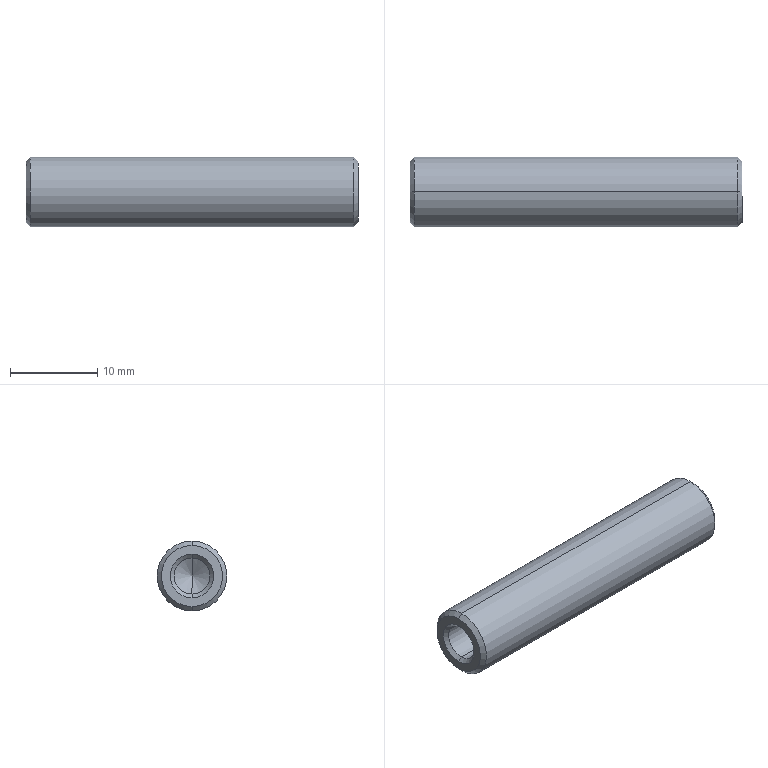Component | SolidWorks | MHF04-D8-L38.stp-1 | 1 solid | 20 faces | box 38 x 8 x 8 mm | volume 1481 mm3 | cone 12 | cylinder 6 | plane 2 | commonest cylinder face diameters 4.134 x4 8 x2
STEP:
#1=CARTESIAN_POINT('',(0.1007,3.568,-1.181));
#2=VERTEX_POINT('',#1);
#3=CARTESIAN_POINT('',(0.1476,3.568,-1.262));
#4=VERTEX_POINT('',#3);
#5=CARTESIAN_POINT('',(0.1476,3.568,-1.262));
#6=DIRECTION('',(0.5,0.,-0.866));
#7=VECTOR('',#6,39.37);
#8=LINE('',#5,#7);
#9=EDGE_CURVE('',#2,#4,#8,.T.);
#10=ORIENTED_EDGE('',*,*,#9,.F.);
#11=CARTESIAN_POINT('',(0.1476,3.568,-1.1));
#12=VERTEX_POINT('',#11);
#13=CARTESIAN_POINT('',(0.1476,3.568,-1.1));
#14=DIRECTION('',(0.5,-0.,0.866));
#15=VECTOR('',#14,39.37);
#16=LINE('',#13,#15);
#17=EDGE_CURVE('',#2,#12,#16,.T.);
#18=ORIENTED_EDGE('',*,*,#17,.T.);
#19=CARTESIAN_POINT('',(0.1476,3.568,-1.181));
#20=DIRECTION('',(1.,0.,0.));
#21=DIRECTION('',(0.,0.,-1.));
#22=AXIS2_PLACEMENT_3D('',#19,#20,#21);
#23=CIRCLE('',#22,0.08138);
#24=EDGE_CURVE('',#12,#4,#23,.T.);
#25=ORIENTED_EDGE('',*,*,#24,.T.);
#26=EDGE_LOOP('',(#10,#18,#25));
#27=FACE_OUTER_BOUND('',#26,.T.);
#28=CARTESIAN_POINT('',(0.1476,3.568,-1.181));
#29=DIRECTION('',(1.,0.,0.));
#30=DIRECTION('',(0.,0.,-1.));
#31=AXIS2_PLACEMENT_3D('',#28,#29,#30);
#32=CONICAL_SURFACE('',#31,0.08138,1.047);
#33=ADVANCED_FACE('',(#27),#32,.F.);
#34=CARTESIAN_POINT('',(0.731,3.568,-1.262));
#35=VERTEX_POINT('',#34);
#36=CARTESIAN_POINT('',(0.731,3.568,-1.1));
#37=VERTEX_POINT('',#36);
#38=CARTESIAN_POINT('',(0.731,3.568,-1.181));
#39=DIRECTION('',(1.,0.,0.));
#40=DIRECTION('',(0.,0.,-1.));
#41=AXIS2_PLACEMENT_3D('',#38,#39,#40);
#42=CIRCLE('',#41,0.08138);
#43=EDGE_CURVE('',#35,#37,#42,.T.);
#44=ORIENTED_EDGE('',*,*,#43,.T.);
#45=CARTESIAN_POINT('',(0.748,3.568,-1.1));
#46=DIRECTION('',(-1.,-0.,-0.));
#47=VECTOR('',#46,39.37);
#48=LINE('',#45,#47);
#49=EDGE_CURVE('',#37,#12,#48,.T.);
#50=ORIENTED_EDGE('',*,*,#49,.T.);
#51=CARTESIAN_POINT('',(0.1476,3.568,-1.181));
#52=DIRECTION('',(1.,0.,0.));
#53=DIRECTION('',(0.,0.,-1.));
#54=AXIS2_PLACEMENT_3D('',#51,#52,#53);
#55=CIRCLE('',#54,0.08138);
#56=EDGE_CURVE('',#4,#12,#55,.T.);
#57=ORIENTED_EDGE('',*,*,#56,.F.);
#58=CARTESIAN_POINT('',(0.748,3.568,-1.262));
#59=DIRECTION('',(-1.,-0.,-0.));
#60=VECTOR('',#59,39.37);
#61=LINE('',#58,#60);
#62=EDGE_CURVE('',#35,#4,#61,.T.);
#63=ORIENTED_EDGE('',*,*,#62,.F.);
#64=EDGE_LOOP('',(#44,#50,#57,#63));
#65=FACE_OUTER_BOUND('',#64,.T.);
#66=CARTESIAN_POINT('',(0.748,3.568,-1.181));
#67=DIRECTION('',(-1.,-0.,-0.));
#68=DIRECTION('',(0.,0.,-1.));
#69=AXIS2_PLACEMENT_3D('',#66,#67,#68);
#70=CYLINDRICAL_SURFACE('',#69,0.08138);
#71=ADVANCED_FACE('',(#65),#70,.F.);
#72=CARTESIAN_POINT('',(0.731,3.568,-1.181));
#73=DIRECTION('',(1.,0.,0.));
#74=DIRECTION('',(0.,0.,-1.));
#75=AXIS2_PLACEMENT_3D('',#72,#73,#74);
#76=CIRCLE('',#75,0.08138);
#77=EDGE_CURVE('',#37,#35,#76,.T.);
#78=ORIENTED_EDGE('',*,*,#77,.F.);
#79=CARTESIAN_POINT('',(0.748,3.568,-1.083));
#80=VERTEX_POINT('',#79);
#81=CARTESIAN_POINT('',(0.748,3.568,-1.083));
#82=DIRECTION('',(0.7071,0.,0.7071));
#83=VECTOR('',#82,39.37);
#84=LINE('',#81,#83);
#85=EDGE_CURVE('',#37,#80,#84,.T.);
#86=ORIENTED_EDGE('',*,*,#85,.T.);
#87=CARTESIAN_POINT('',(0.748,3.568,-1.28));
#88=VERTEX_POINT('',#87);
#89=CARTESIAN_POINT('',(0.748,3.568,-1.181));
#90=DIRECTION('',(1.,0.,0.));
#91=DIRECTION('',(0.,0.,-1.));
#92=AXIS2_PLACEMENT_3D('',#89,#90,#91);
#93=CIRCLE('',#92,0.09843);
#94=EDGE_CURVE('',#80,#88,#93,.T.);
#95=ORIENTED_EDGE('',*,*,#94,.T.);
#96=CARTESIAN_POINT('',(0.748,3.568,-1.28));
#97=DIRECTION('',(0.7071,0.,-0.7071));
#98=VECTOR('',#97,39.37);
#99=LINE('',#96,#98);
#100=EDGE_CURVE('',#35,#88,#99,.T.);
#101=ORIENTED_EDGE('',*,*,#100,.F.);
#102=EDGE_LOOP('',(#78,#86,#95,#101));
#103=FACE_OUTER_BOUND('',#102,.T.);
#104=CARTESIAN_POINT('',(0.748,3.568,-1.181));
#105=DIRECTION('',(1.,0.,0.));
#106=DIRECTION('',(0.,0.,-1.));
#107=AXIS2_PLACEMENT_3D('',#104,#105,#106);
#108=CONICAL_SURFACE('',#107,0.09843,0.7854);
#109=ADVANCED_FACE('',(#103),#108,.F.);
#110=CARTESIAN_POINT('',(0.748,3.568,-1.319));
#111=VERTEX_POINT('',#110);
#112=CARTESIAN_POINT('',(0.748,3.568,-1.043));
#113=VERTEX_POINT('',#112);
#114=CARTESIAN_POINT('',(0.748,3.568,-1.181));
#115=DIRECTION('',(1.,0.,0.));
#116=DIRECTION('',(0.,0.,-1.));
#117=AXIS2_PLACEMENT_3D('',#114,#115,#116);
#118=CIRCLE('',#117,0.1378);
#119=EDGE_CURVE('',#111,#113,#118,.T.);
#120=ORIENTED_EDGE('',*,*,#119,.F.);
#121=CARTESIAN_POINT('',(0.7283,3.568,-1.339));
#122=VERTEX_POINT('',#121);
#123=CARTESIAN_POINT('',(0.7283,3.568,-1.339));
#124=DIRECTION('',(-0.7071,0.,-0.7071));
#125=VECTOR('',#124,39.37);
#126=LINE('',#123,#125);
#127=EDGE_CURVE('',#111,#122,#126,.T.);
#128=ORIENTED_EDGE('',*,*,#127,.T.);
#129=CARTESIAN_POINT('',(0.7283,3.568,-1.024));
#130=VERTEX_POINT('',#129);
#131=CARTESIAN_POINT('',(0.7283,3.568,-1.181));
#132=DIRECTION('',(1.,0.,0.));
#133=DIRECTION('',(0.,0.,-1.));
#134=AXIS2_PLACEMENT_3D('',#131,#132,#133);
#135=CIRCLE('',#134,0.1575);
#136=EDGE_CURVE('',#122,#130,#135,.T.);
#137=ORIENTED_EDGE('',*,*,#136,.T.);
#138=CARTESIAN_POINT('',(0.7283,3.568,-1.024));
#139=DIRECTION('',(-0.7071,-0.,0.7071));
#140=VECTOR('',#139,39.37);
#141=LINE('',#138,#140);
#142=EDGE_CURVE('',#113,#130,#141,.T.);
#143=ORIENTED_EDGE('',*,*,#142,.F.);
#144=EDGE_LOOP('',(#120,#128,#137,#143));
#145=FACE_OUTER_BOUND('',#144,.T.);
#146=CARTESIAN_POINT('',(0.7283,3.568,-1.181));
#147=DIRECTION('',(-1.,-0.,-0.));
#148=DIRECTION('',(0.,0.,1.));
#149=AXIS2_PLACEMENT_3D('',#146,#147,#148);
#150=CONICAL_SURFACE('',#149,0.1575,0.7854);
#151=ADVANCED_FACE('',(#145),#150,.T.);
#152=CARTESIAN_POINT('',(0.7283,3.568,-1.181));
#153=DIRECTION('',(1.,0.,0.));
#154=DIRECTION('',(0.,0.,-1.));
#155=AXIS2_PLACEMENT_3D('',#152,#153,#154);
#156=CIRCLE('',#155,0.1575);
#157=EDGE_CURVE('',#130,#122,#156,.T.);
#158=ORIENTED_EDGE('',*,*,#157,.F.);
#159=CARTESIAN_POINT('',(-0.7283,3.568,-1.024));
#160=VERTEX_POINT('',#159);
#161=CARTESIAN_POINT('',(0.748,3.568,-1.024));
#162=DIRECTION('',(-1.,-0.,-0.));
#163=VECTOR('',#162,39.37);
#164=LINE('',#161,#163);
#165=EDGE_CURVE('',#130,#160,#164,.T.);
#166=ORIENTED_EDGE('',*,*,#165,.T.);
#167=CARTESIAN_POINT('',(-0.7283,3.568,-1.339));
#168=VERTEX_POINT('',#167);
#169=CARTESIAN_POINT('',(-0.7283,3.568,-1.181));
#170=DIRECTION('',(1.,0.,0.));
#171=DIRECTION('',(0.,0.,-1.));
#172=AXIS2_PLACEMENT_3D('',#169,#170,#171);
#173=CIRCLE('',#172,0.1575);
#174=EDGE_CURVE('',#160,#168,#173,.T.);
#175=ORIENTED_EDGE('',*,*,#174,.T.);
#176=CARTESIAN_POINT('',(0.748,3.568,-1.339));
#177=DIRECTION('',(-1.,-0.,-0.));
#178=VECTOR('',#177,39.37);
#179=LINE('',#176,#178);
#180=EDGE_CURVE('',#122,#168,#179,.T.);
#181=ORIENTED_EDGE('',*,*,#180,.F.);
#182=EDGE_LOOP('',(#158,#166,#175,#181));
#183=FACE_OUTER_BOUND('',#182,.T.);
#184=CARTESIAN_POINT('',(0.748,3.568,-1.181));
#185=DIRECTION('',(-1.,-0.,-0.));
#186=DIRECTION('',(0.,0.,-1.));
#187=AXIS2_PLACEMENT_3D('',#184,#185,#186);
#188=CYLINDRICAL_SURFACE('',#187,0.1575);
#189=ADVANCED_FACE('',(#183),#188,.T.);
#190=CARTESIAN_POINT('',(-0.748,3.568,-1.319));
#191=VERTEX_POINT('',#190);
#192=CARTESIAN_POINT('',(-0.748,3.568,-1.043));
#193=VERTEX_POINT('',#192);
#194=CARTESIAN_POINT('',(-0.748,3.568,-1.181));
#195=DIRECTION('',(1.,0.,0.));
#196=DIRECTION('',(0.,0.,-1.));
#197=AXIS2_PLACEMENT_3D('',#194,#195,#196);
#198=CIRCLE('',#197,0.1378);
#199=EDGE_CURVE('',#191,#193,#198,.T.);
#200=ORIENTED_EDGE('',*,*,#199,.T.);
#201=CARTESIAN_POINT('',(-0.748,3.568,-1.043));
#202=DIRECTION('',(0.7071,0.,0.7071));
#203=VECTOR('',#202,39.37);
#204=LINE('',#201,#203);
#205=EDGE_CURVE('',#193,#160,#204,.T.);
#206=ORIENTED_EDGE('',*,*,#205,.T.);
#207=CARTESIAN_POINT('',(-0.7283,3.568,-1.181));
#208=DIRECTION('',(1.,0.,0.));
#209=DIRECTION('',(0.,0.,-1.));
#210=AXIS2_PLACEMENT_3D('',#207,#208,#209);
#211=CIRCLE('',#210,0.1575);
#212=EDGE_CURVE('',#168,#160,#211,.T.);
#213=ORIENTED_EDGE('',*,*,#212,.F.);
#214=CARTESIAN_POINT('',(-0.748,3.568,-1.319));
#215=DIRECTION('',(0.7071,0.,-0.7071));
#216=VECTOR('',#215,39.37);
#217=LINE('',#214,#216);
#218=EDGE_CURVE('',#191,#168,#217,.T.);
#219=ORIENTED_EDGE('',*,*,#218,.F.);
#220=EDGE_LOOP('',(#200,#206,#213,#219));
#221=FACE_OUTER_BOUND('',#220,.T.);
#222=CARTESIAN_POINT('',(-0.748,3.568,-1.181));
#223=DIRECTION('',(1.,0.,0.));
#224=DIRECTION('',(0.,0.,-1.));
#225=AXIS2_PLACEMENT_3D('',#222,#223,#224);
#226=CONICAL_SURFACE('',#225,0.1378,0.7854);
#227=ADVANCED_FACE('',(#221),#226,.T.);
#228=CARTESIAN_POINT('',(-0.731,3.568,-1.1));
#229=VERTEX_POINT('',#228);
#230=CARTESIAN_POINT('',(-0.731,3.568,-1.262));
#231=VERTEX_POINT('',#230);
#232=CARTESIAN_POINT('',(-0.731,3.568,-1.181));
#233=DIRECTION('',(1.,0.,0.));
#234=DIRECTION('',(0.,0.,-1.));
#235=AXIS2_PLACEMENT_3D('',#232,#233,#234);
#236=CIRCLE('',#235,0.08138);
#237=EDGE_CURVE('',#229,#231,#236,.T.);
#238=ORIENTED_EDGE('',*,*,#237,.T.);
#239=CARTESIAN_POINT('',(-0.748,3.568,-1.28));
#240=VERTEX_POINT('',#239);
#241=CARTESIAN_POINT('',(-0.731,3.568,-1.262));
#242=DIRECTION('',(-0.7071,0.,-0.7071));
#243=VECTOR('',#242,39.37);
#244=LINE('',#241,#243);
#245=EDGE_CURVE('',#231,#240,#244,.T.);
#246=ORIENTED_EDGE('',*,*,#245,.T.);
#247=CARTESIAN_POINT('',(-0.748,3.568,-1.083));
#248=VERTEX_POINT('',#247);
#249=CARTESIAN_POINT('',(-0.748,3.568,-1.181));
#250=DIRECTION('',(1.,0.,0.));
#251=DIRECTION('',(0.,0.,-1.));
#252=AXIS2_PLACEMENT_3D('',#249,#250,#251);
#253=CIRCLE('',#252,0.09843);
#254=EDGE_CURVE('',#248,#240,#253,.T.);
#255=ORIENTED_EDGE('',*,*,#254,.F.);
#256=CARTESIAN_POINT('',(-0.731,3.568,-1.1));
#257=DIRECTION('',(-0.7071,-0.,0.7071));
#258=VECTOR('',#257,39.37);
#259=LINE('',#256,#258);
#260=EDGE_CURVE('',#229,#248,#259,.T.);
#261=ORIENTED_EDGE('',*,*,#260,.F.);
#262=EDGE_LOOP('',(#238,#246,#255,#261));
#263=FACE_OUTER_BOUND('',#262,.T.);
#264=CARTESIAN_POINT('',(-0.731,3.568,-1.181));
#265=DIRECTION('',(-1.,-0.,-0.));
#266=DIRECTION('',(0.,0.,1.));
#267=AXIS2_PLACEMENT_3D('',#264,#265,#266);
#268=CONICAL_SURFACE('',#267,0.08138,0.7854);
#269=ADVANCED_FACE('',(#263),#268,.F.);
#270=CARTESIAN_POINT('',(-0.1476,3.568,-1.262));
#271=VERTEX_POINT('',#270);
#272=CARTESIAN_POINT('',(-0.1476,3.568,-1.1));
#273=VERTEX_POINT('',#272);
#274=CARTESIAN_POINT('',(-0.1476,3.568,-1.181));
#275=DIRECTION('',(1.,0.,0.));
#276=DIRECTION('',(0.,0.,-1.));
#277=AXIS2_PLACEMENT_3D('',#274,#275,#276);
#278=CIRCLE('',#277,0.08138);
#279=EDGE_CURVE('',#271,#273,#278,.T.);
#280=ORIENTED_EDGE('',*,*,#279,.T.);
#281=CARTESIAN_POINT('',(0.748,3.568,-1.1));
#282=DIRECTION('',(-1.,-0.,-0.));
#283=VECTOR('',#282,39.37);
#284=LINE('',#281,#283);
#285=EDGE_CURVE('',#273,#229,#284,.T.);
#286=ORIENTED_EDGE('',*,*,#285,.T.);
#287=CARTESIAN_POINT('',(-0.731,3.568,-1.181));
#288=DIRECTION('',(1.,0.,0.));
#289=DIRECTION('',(0.,0.,-1.));
#290=AXIS2_PLACEMENT_3D('',#287,#288,#289);
#291=CIRCLE('',#290,0.08138);
#292=EDGE_CURVE('',#231,#229,#291,.T.);
#293=ORIENTED_EDGE('',*,*,#292,.F.);
#294=CARTESIAN_POINT('',(0.748,3.568,-1.262));
#295=DIRECTION('',(-1.,-0.,-0.));
#296=VECTOR('',#295,39.37);
#297=LINE('',#294,#296);
#298=EDGE_CURVE('',#271,#231,#297,.T.);
#299=ORIENTED_EDGE('',*,*,#298,.F.);
#300=EDGE_LOOP('',(#280,#286,#293,#299));
#301=FACE_OUTER_BOUND('',#300,.T.);
#302=CARTESIAN_POINT('',(0.748,3.568,-1.181));
#303=DIRECTION('',(-1.,-0.,-0.));
#304=DIRECTION('',(0.,0.,-1.));
#305=AXIS2_PLACEMENT_3D('',#302,#303,#304);
#306=CYLINDRICAL_SURFACE('',#305,0.08138);
#307=ADVANCED_FACE('',(#301),#306,.F.);
#308=CARTESIAN_POINT('',(-0.1007,3.568,-1.181));
#309=VERTEX_POINT('',#308);
#310=CARTESIAN_POINT('',(-19.786,3.568,32.914));
#311=DIRECTION('',(-0.5,-0.,0.866));
#312=VECTOR('',#311,39.37);
#313=LINE('',#310,#312);
#314=EDGE_CURVE('',#309,#273,#313,.T.);
#315=ORIENTED_EDGE('',*,*,#314,.F.);
#316=CARTESIAN_POINT('',(-19.786,3.568,-35.277));
#317=DIRECTION('',(-0.5,0.,-0.866));
#318=VECTOR('',#317,39.37);
#319=LINE('',#316,#318);
#320=EDGE_CURVE('',#309,#271,#319,.T.);
#321=ORIENTED_EDGE('',*,*,#320,.T.);
#322=CARTESIAN_POINT('',(-0.1476,3.568,-1.181));
#323=DIRECTION('',(1.,0.,0.));
#324=DIRECTION('',(0.,0.,-1.));
#325=AXIS2_PLACEMENT_3D('',#322,#323,#324);
#326=CIRCLE('',#325,0.08138);
#327=EDGE_CURVE('',#273,#271,#326,.T.);
#328=ORIENTED_EDGE('',*,*,#327,.F.);
#329=EDGE_LOOP('',(#315,#321,#328));
#330=FACE_OUTER_BOUND('',#329,.T.);
#331=CARTESIAN_POINT('',(-19.786,3.568,-1.181));
#332=DIRECTION('',(-1.,-0.,-0.));
#333=DIRECTION('',(-0.,-0.,1.));
#334=AXIS2_PLACEMENT_3D('',#331,#332,#333);
#335=CONICAL_SURFACE('',#334,34.095,1.047);
#336=ADVANCED_FACE('',(#330),#335,.F.);
#337=ORIENTED_EDGE('',*,*,#320,.F.);
#338=ORIENTED_EDGE('',*,*,#314,.T.);
#339=ORIENTED_EDGE('',*,*,#279,.F.);
#340=EDGE_LOOP('',(#337,#338,#339));
#341=FACE_OUTER_BOUND('',#340,.T.);
#342=CARTESIAN_POINT('',(-19.786,3.568,-1.181));
#343=DIRECTION('',(-1.,-0.,-0.));
#344=DIRECTION('',(-0.,-0.,1.));
#345=AXIS2_PLACEMENT_3D('',#342,#343,#344);
#346=CONICAL_SURFACE('',#345,34.095,1.047);
#347=ADVANCED_FACE('',(#341),#346,.F.);
#348=ORIENTED_EDGE('',*,*,#285,.F.);
#349=ORIENTED_EDGE('',*,*,#327,.T.);
#350=ORIENTED_EDGE('',*,*,#298,.T.);
#351=ORIENTED_EDGE('',*,*,#237,.F.);
#352=EDGE_LOOP('',(#348,#349,#350,#351));
#353=FACE_OUTER_BOUND('',#352,.T.);
#354=CARTESIAN_POINT('',(0.748,3.568,-1.181));
#355=DIRECTION('',(-1.,-0.,-0.));
#356=DIRECTION('',(0.,0.,-1.));
#357=AXIS2_PLACEMENT_3D('',#354,#355,#356);
#358=CYLINDRICAL_SURFACE('',#357,0.08138);
#359=ADVANCED_FACE('',(#353),#358,.F.);
#360=ORIENTED_EDGE('',*,*,#245,.F.);
#361=ORIENTED_EDGE('',*,*,#292,.T.);
#362=ORIENTED_EDGE('',*,*,#260,.T.);
#363=CARTESIAN_POINT('',(-0.748,3.568,-1.181));
#364=DIRECTION('',(1.,0.,0.));
#365=DIRECTION('',(0.,0.,-1.));
#366=AXIS2_PLACEMENT_3D('',#363,#364,#365);
#367=CIRCLE('',#366,0.09843);
#368=EDGE_CURVE('',#240,#248,#367,.T.);
#369=ORIENTED_EDGE('',*,*,#368,.F.);
#370=EDGE_LOOP('',(#360,#361,#362,#369));
#371=FACE_OUTER_BOUND('',#370,.T.);
#372=CARTESIAN_POINT('',(-0.731,3.568,-1.181));
#373=DIRECTION('',(-1.,-0.,-0.));
#374=DIRECTION('',(0.,0.,1.));
#375=AXIS2_PLACEMENT_3D('',#372,#373,#374);
#376=CONICAL_SURFACE('',#375,0.08138,0.7854);
#377=ADVANCED_FACE('',(#371),#376,.F.);
#378=ORIENTED_EDGE('',*,*,#199,.F.);
#379=CARTESIAN_POINT('',(-0.748,3.568,-1.181));
#380=DIRECTION('',(1.,0.,0.));
#381=DIRECTION('',(0.,0.,-1.));
#382=AXIS2_PLACEMENT_3D('',#379,#380,#381);
#383=CIRCLE('',#382,0.1378);
#384=EDGE_CURVE('',#193,#191,#383,.T.);
#385=ORIENTED_EDGE('',*,*,#384,.F.);
#386=EDGE_LOOP('',(#378,#385));
#387=FACE_OUTER_BOUND('',#386,.T.);
#388=ORIENTED_EDGE('',*,*,#254,.T.);
#389=ORIENTED_EDGE('',*,*,#368,.T.);
#390=EDGE_LOOP('',(#388,#389));
#391=FACE_BOUND('',#390,.T.);
#392=CARTESIAN_POINT('',(-0.748,3.666,-1.181));
#393=DIRECTION('',(1.,0.,0.));
#394=DIRECTION('',(0.,-1.,-0.));
#395=AXIS2_PLACEMENT_3D('',#392,#393,#394);
#396=PLANE('',#395);
#397=ADVANCED_FACE('',(#387,#391),#396,.F.);
#398=ORIENTED_EDGE('',*,*,#205,.F.);
#399=ORIENTED_EDGE('',*,*,#384,.T.);
#400=ORIENTED_EDGE('',*,*,#218,.T.);
#401=ORIENTED_EDGE('',*,*,#174,.F.);
#402=EDGE_LOOP('',(#398,#399,#400,#401));
#403=FACE_OUTER_BOUND('',#402,.T.);
#404=CARTESIAN_POINT('',(-0.748,3.568,-1.181));
#405=DIRECTION('',(1.,0.,0.));
#406=DIRECTION('',(0.,0.,-1.));
#407=AXIS2_PLACEMENT_3D('',#404,#405,#406);
#408=CONICAL_SURFACE('',#407,0.1378,0.7854);
#409=ADVANCED_FACE('',(#403),#408,.T.);
#410=ORIENTED_EDGE('',*,*,#165,.F.);
#411=ORIENTED_EDGE('',*,*,#136,.F.);
#412=ORIENTED_EDGE('',*,*,#180,.T.);
#413=ORIENTED_EDGE('',*,*,#212,.T.);
#414=EDGE_LOOP('',(#410,#411,#412,#413));
#415=FACE_OUTER_BOUND('',#414,.T.);
#416=CARTESIAN_POINT('',(0.748,3.568,-1.181));
#417=DIRECTION('',(-1.,-0.,-0.));
#418=DIRECTION('',(0.,0.,-1.));
#419=AXIS2_PLACEMENT_3D('',#416,#417,#418);
#420=CYLINDRICAL_SURFACE('',#419,0.1575);
#421=ADVANCED_FACE('',(#415),#420,.T.);
#422=ORIENTED_EDGE('',*,*,#127,.F.);
#423=CARTESIAN_POINT('',(0.748,3.568,-1.181));
#424=DIRECTION('',(1.,0.,0.));
#425=DIRECTION('',(0.,0.,-1.));
#426=AXIS2_PLACEMENT_3D('',#423,#424,#425);
#427=CIRCLE('',#426,0.1378);
#428=EDGE_CURVE('',#113,#111,#427,.T.);
#429=ORIENTED_EDGE('',*,*,#428,.F.);
#430=ORIENTED_EDGE('',*,*,#142,.T.);
#431=ORIENTED_EDGE('',*,*,#157,.T.);
#432=EDGE_LOOP('',(#422,#429,#430,#431));
#433=FACE_OUTER_BOUND('',#432,.T.);
#434=CARTESIAN_POINT('',(0.7283,3.568,-1.181));
#435=DIRECTION('',(-1.,-0.,-0.));
#436=DIRECTION('',(0.,0.,1.));
#437=AXIS2_PLACEMENT_3D('',#434,#435,#436);
#438=CONICAL_SURFACE('',#437,0.1575,0.7854);
#439=ADVANCED_FACE('',(#433),#438,.T.);
#440=ORIENTED_EDGE('',*,*,#428,.T.);
#441=ORIENTED_EDGE('',*,*,#119,.T.);
#442=EDGE_LOOP('',(#440,#441));
#443=FACE_OUTER_BOUND('',#442,.T.);
#444=CARTESIAN_POINT('',(0.748,3.568,-1.181));
#445=DIRECTION('',(1.,0.,0.));
#446=DIRECTION('',(0.,0.,-1.));
#447=AXIS2_PLACEMENT_3D('',#444,#445,#446);
#448=CIRCLE('',#447,0.09843);
#449=EDGE_CURVE('',#88,#80,#448,.T.);
#450=ORIENTED_EDGE('',*,*,#449,.F.);
#451=ORIENTED_EDGE('',*,*,#94,.F.);
#452=EDGE_LOOP('',(#450,#451));
#453=FACE_BOUND('',#452,.T.);
#454=CARTESIAN_POINT('',(0.748,3.705,-1.181));
#455=DIRECTION('',(-1.,-0.,-0.));
#456=DIRECTION('',(-0.,-0.,1.));
#457=AXIS2_PLACEMENT_3D('',#454,#455,#456);
#458=PLANE('',#457);
#459=ADVANCED_FACE('',(#443,#453),#458,.F.);
#460=ORIENTED_EDGE('',*,*,#85,.F.);
#461=ORIENTED_EDGE('',*,*,#43,.F.);
#462=ORIENTED_EDGE('',*,*,#100,.T.);
#463=ORIENTED_EDGE('',*,*,#449,.T.);
#464=EDGE_LOOP('',(#460,#461,#462,#463));
#465=FACE_OUTER_BOUND('',#464,.T.);
#466=CARTESIAN_POINT('',(0.748,3.568,-1.181));
#467=DIRECTION('',(1.,0.,0.));
#468=DIRECTION('',(0.,0.,-1.));
#469=AXIS2_PLACEMENT_3D('',#466,#467,#468);
#470=CONICAL_SURFACE('',#469,0.09843,0.7854);
#471=ADVANCED_FACE('',(#465),#470,.F.);
#472=ORIENTED_EDGE('',*,*,#49,.F.);
#473=ORIENTED_EDGE('',*,*,#77,.T.);
#474=ORIENTED_EDGE('',*,*,#62,.T.);
#475=ORIENTED_EDGE('',*,*,#24,.F.);
#476=EDGE_LOOP('',(#472,#473,#474,#475));
#477=FACE_OUTER_BOUND('',#476,.T.);
#478=CARTESIAN_POINT('',(0.748,3.568,-1.181));
#479=DIRECTION('',(-1.,-0.,-0.));
#480=DIRECTION('',(0.,0.,-1.));
#481=AXIS2_PLACEMENT_3D('',#478,#479,#480);
#482=CYLINDRICAL_SURFACE('',#481,0.08138);
#483=ADVANCED_FACE('',(#477),#482,.F.);
#484=ORIENTED_EDGE('',*,*,#17,.F.);
#485=ORIENTED_EDGE('',*,*,#9,.T.);
#486=ORIENTED_EDGE('',*,*,#56,.T.);
#487=EDGE_LOOP('',(#484,#485,#486));
#488=FACE_OUTER_BOUND('',#487,.T.);
#489=CARTESIAN_POINT('',(0.1476,3.568,-1.181));
#490=DIRECTION('',(1.,0.,0.));
#491=DIRECTION('',(0.,0.,-1.));
#492=AXIS2_PLACEMENT_3D('',#489,#490,#491);
#493=CONICAL_SURFACE('',#492,0.08138,1.047);
#494=ADVANCED_FACE('',(#488),#493,.F.);
#495=CLOSED_SHELL('',(#33,#71,#109,#151,#189,#227,#269,#307,#336,#347,#359,#377,#397,#409,#421,#439,#459,#471,#483,#494));
#496=MANIFOLD_SOLID_BREP('',#495);
#497=CARTESIAN_POINT('',(0.,0.,0.));
#498=DIRECTION('',(0.,0.,1.));
#499=DIRECTION('',(1.,0.,0.));
#500=AXIS2_PLACEMENT_3D('',#497,#498,#499);
#501=(LENGTH_UNIT()NAMED_UNIT(*)SI_UNIT($,.METRE.));
#502=LENGTH_MEASURE_WITH_UNIT(LENGTH_MEASURE(0.0254),#501);
#503=DIMENSIONAL_EXPONENTS(1.,0.,0.,0.,0.,0.,0.);
#504=(CONVERSION_BASED_UNIT('',#502)LENGTH_UNIT()NAMED_UNIT(#503));
#505=UNCERTAINTY_MEASURE_WITH_UNIT(LENGTH_MEASURE(0.00001),#504,'','');
#506=(NAMED_UNIT(*)PLANE_ANGLE_UNIT()SI_UNIT($,.RADIAN.));
#507=(NAMED_UNIT(*)SI_UNIT($,.STERADIAN.)SOLID_ANGLE_UNIT());
#508=(GEOMETRIC_REPRESENTATION_CONTEXT(3)GLOBAL_UNCERTAINTY_ASSIGNED_CONTEXT((#505))GLOBAL_UNIT_ASSIGNED_CONTEXT((#504,#506,#507))REPRESENTATION_CONTEXT('',''));
#509=ADVANCED_BREP_SHAPE_REPRESENTATION('',(#496,#500),#508);
#510=COLOUR_RGB('',0.7922,0.8196,0.9333);
#511=FILL_AREA_STYLE_COLOUR('',#510);
#512=FILL_AREA_STYLE('',(#511));
#513=SURFACE_STYLE_FILL_AREA(#512);
#514=SURFACE_SIDE_STYLE('',(#513));
#515=SURFACE_STYLE_USAGE(.BOTH.,#514);
#516=PRESENTATION_STYLE_ASSIGNMENT((#515));
#517=STYLED_ITEM('',(#516),#496);
#518=PRESENTATION_LAYER_ASSIGNMENT('','',(#517));
#519=(LENGTH_UNIT()NAMED_UNIT(*)SI_UNIT($,.METRE.));
#520=LENGTH_MEASURE_WITH_UNIT(LENGTH_MEASURE(0.0254),#519);
#521=DIMENSIONAL_EXPONENTS(1.,0.,0.,0.,0.,0.,0.);
#522=(CONVERSION_BASED_UNIT('',#520)LENGTH_UNIT()NAMED_UNIT(#521));
#523=UNCERTAINTY_MEASURE_WITH_UNIT(LENGTH_MEASURE(0.00001),#522,'','');
#524=(NAMED_UNIT(*)PLANE_ANGLE_UNIT()SI_UNIT($,.RADIAN.));
#525=(NAMED_UNIT(*)SI_UNIT($,.STERADIAN.)SOLID_ANGLE_UNIT());
#526=(GEOMETRIC_REPRESENTATION_CONTEXT(3)GLOBAL_UNCERTAINTY_ASSIGNED_CONTEXT((#523))GLOBAL_UNIT_ASSIGNED_CONTEXT((#522,#524,#525))REPRESENTATION_CONTEXT('',''));
#527=MECHANICAL_DESIGN_GEOMETRIC_PRESENTATION_REPRESENTATION('',(#517),#526);